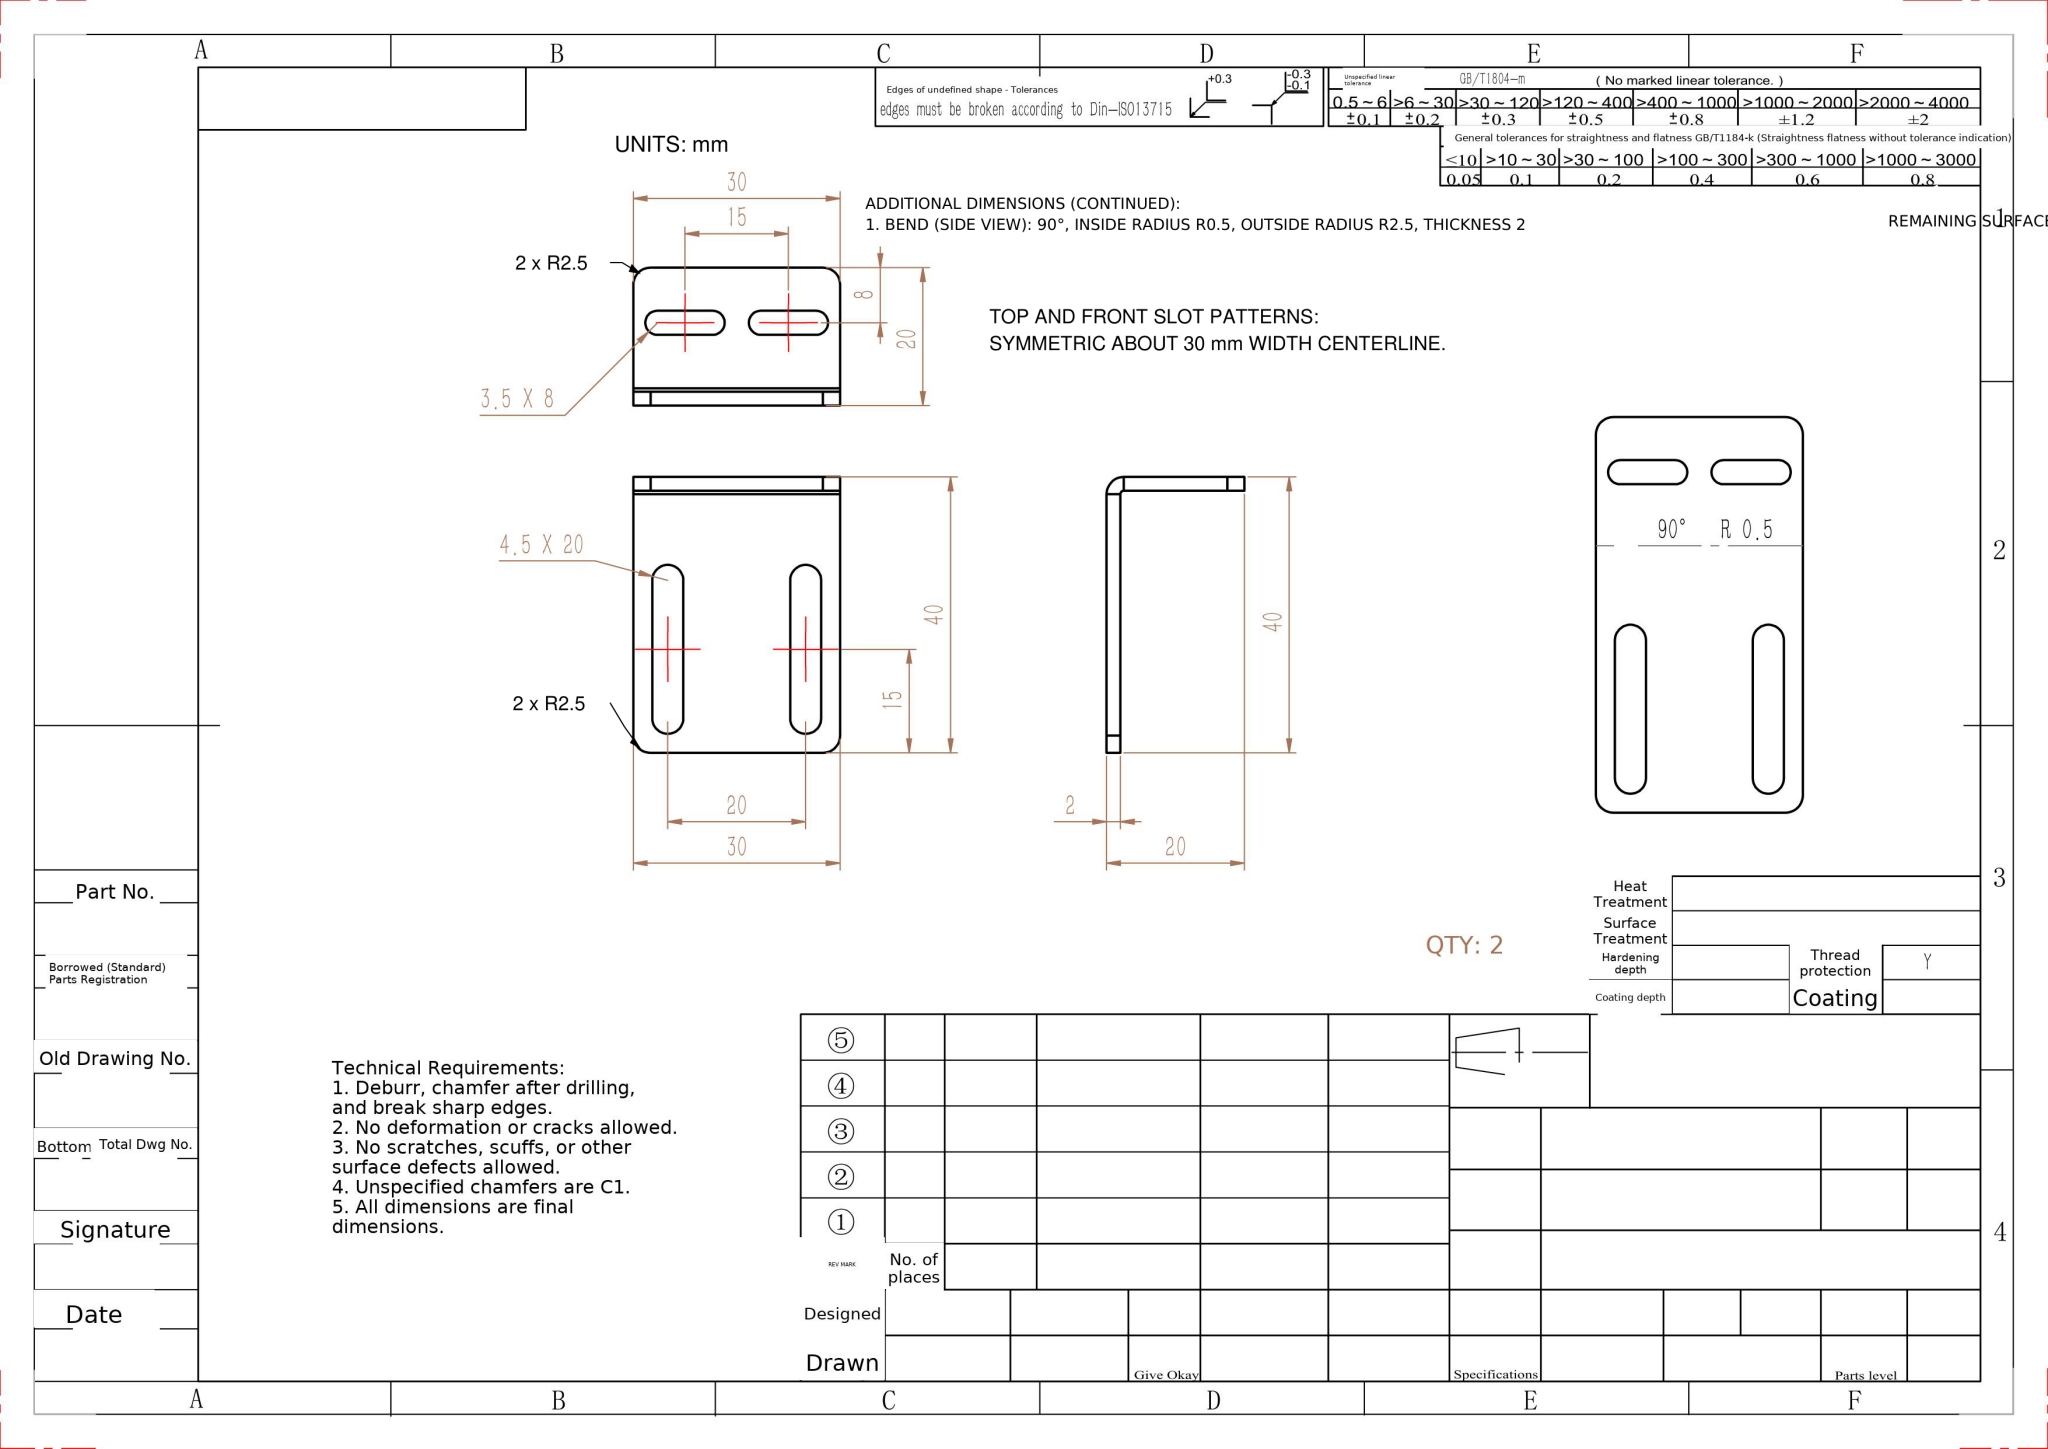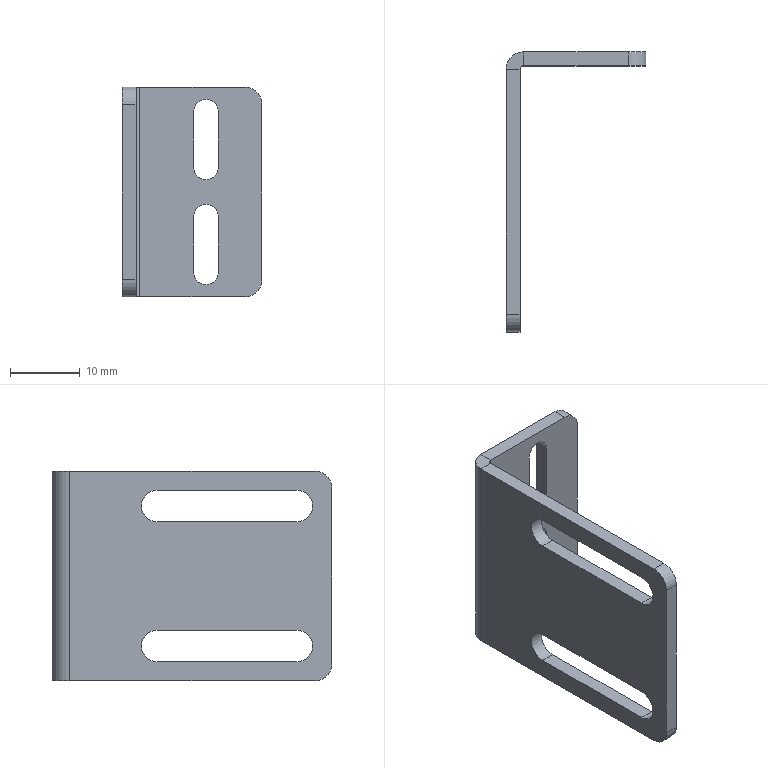Part | NX | mm | 1 solid | 36 faces | box 20 x 40 x 30 mm | volume 2857 mm3 | plane 20 | cylinder 16 | commonest cylinder face diameters 3.5 x6 5 x5 4.5 x4 1 x1